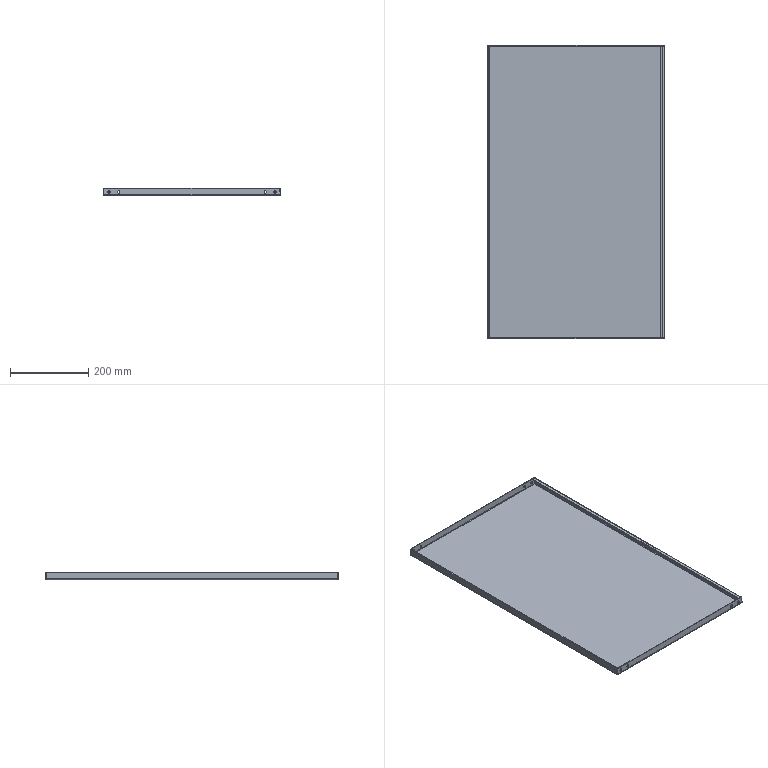Component | SolidWorks | Partition(No.23)-1 | 1 solid | 66 faces | volume 766964 mm3 | plane 40 | cylinder 26 | commonest cylinder face diameters 6.5 x16 6 x5 2 x5 | material Plain Carbon Steel